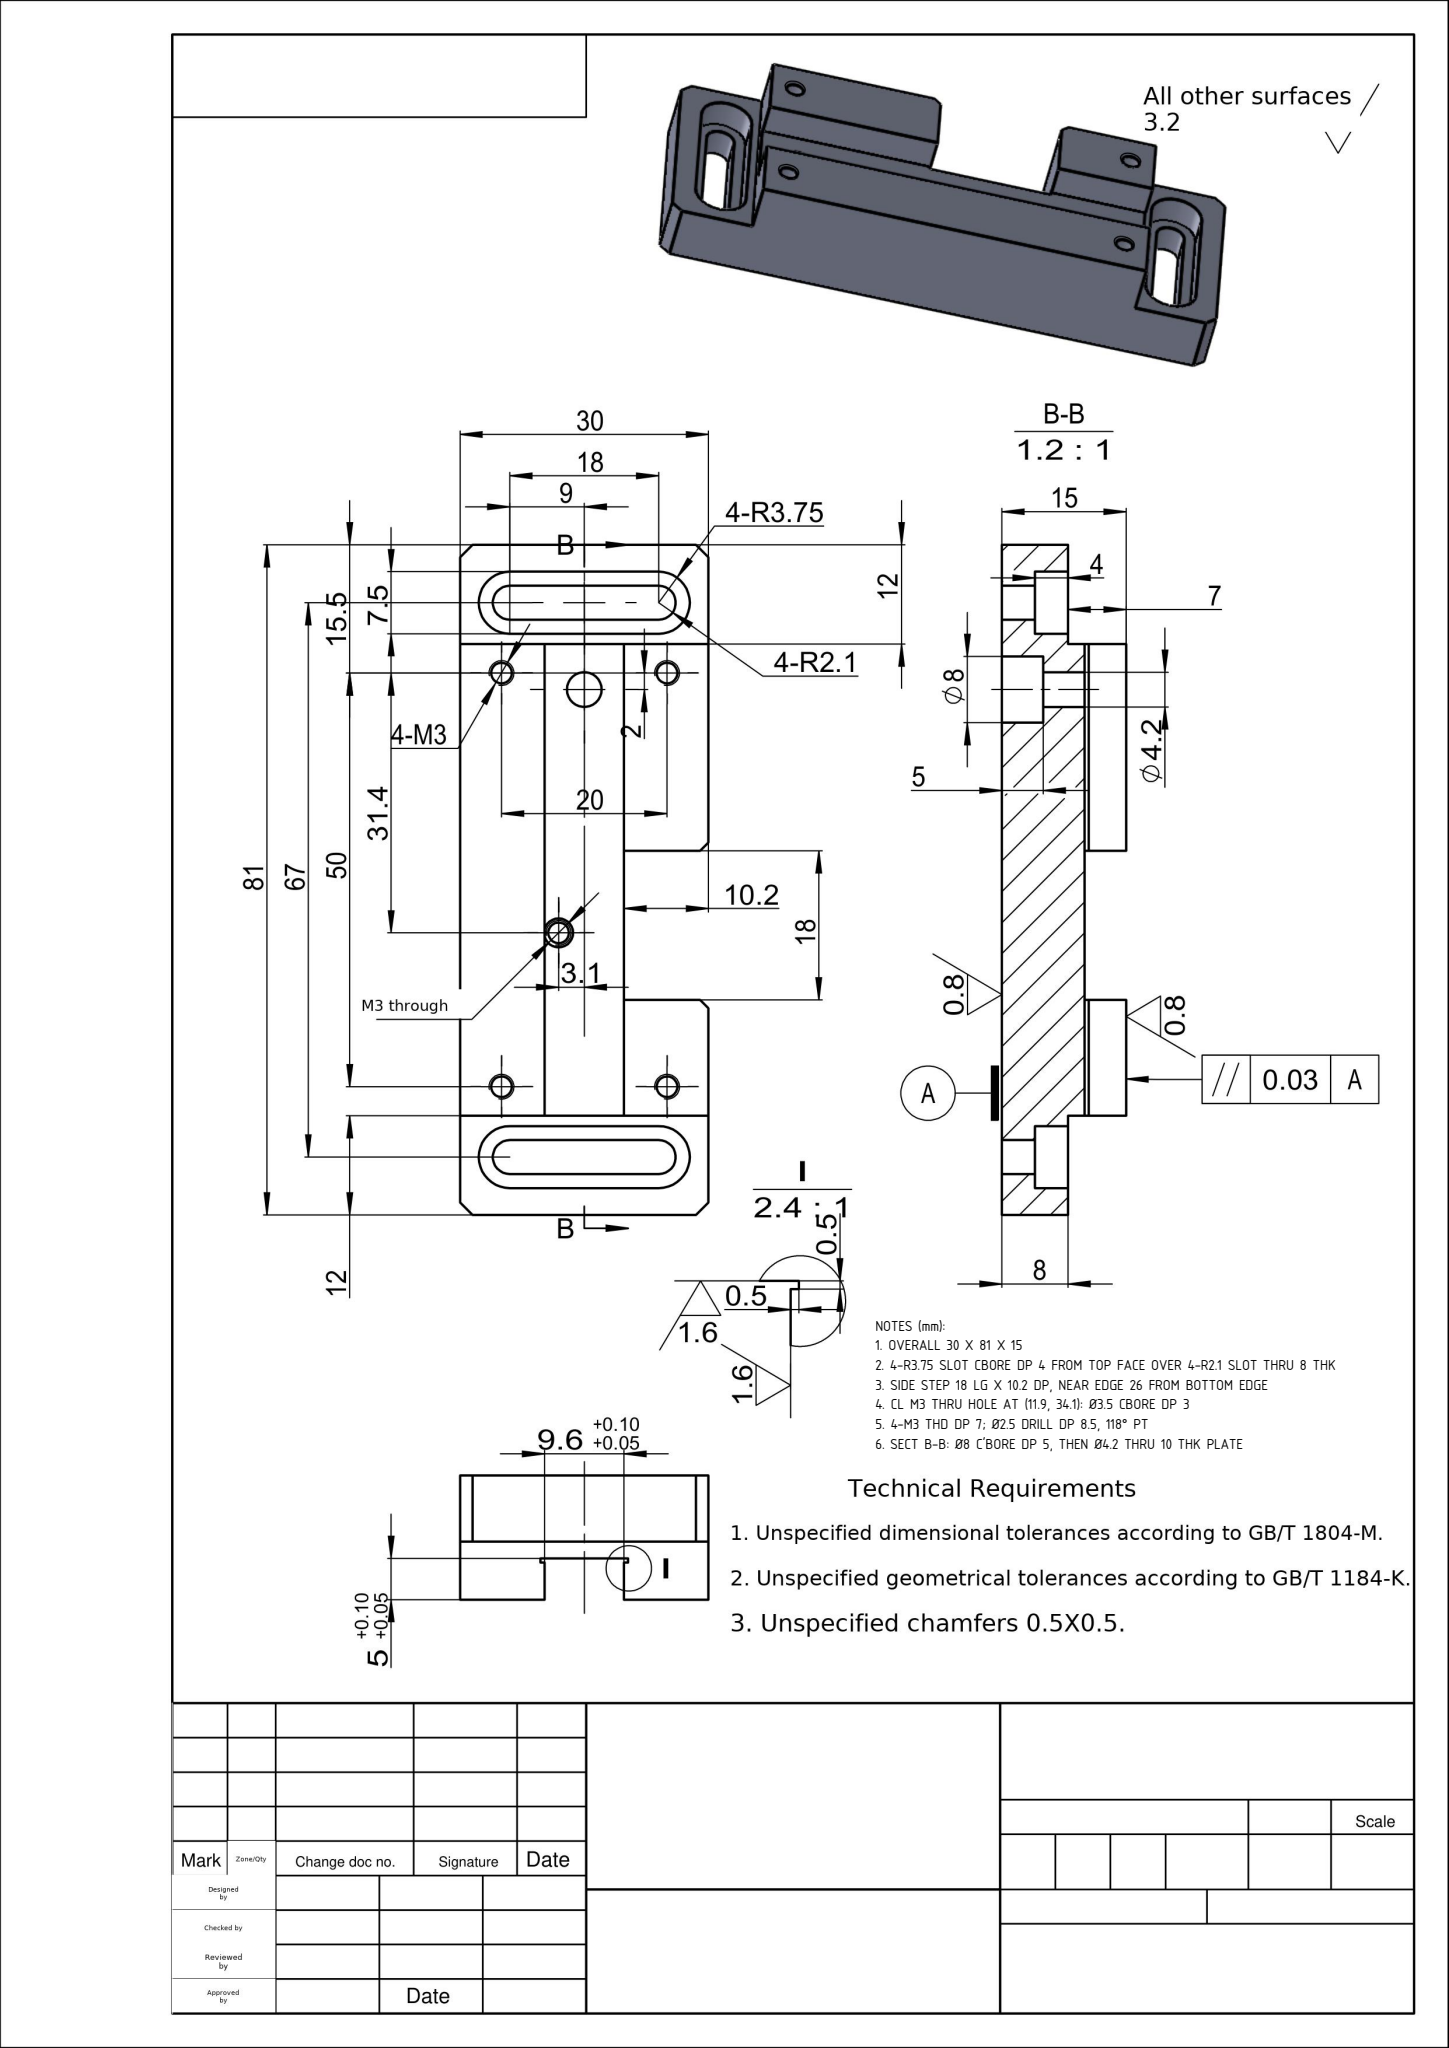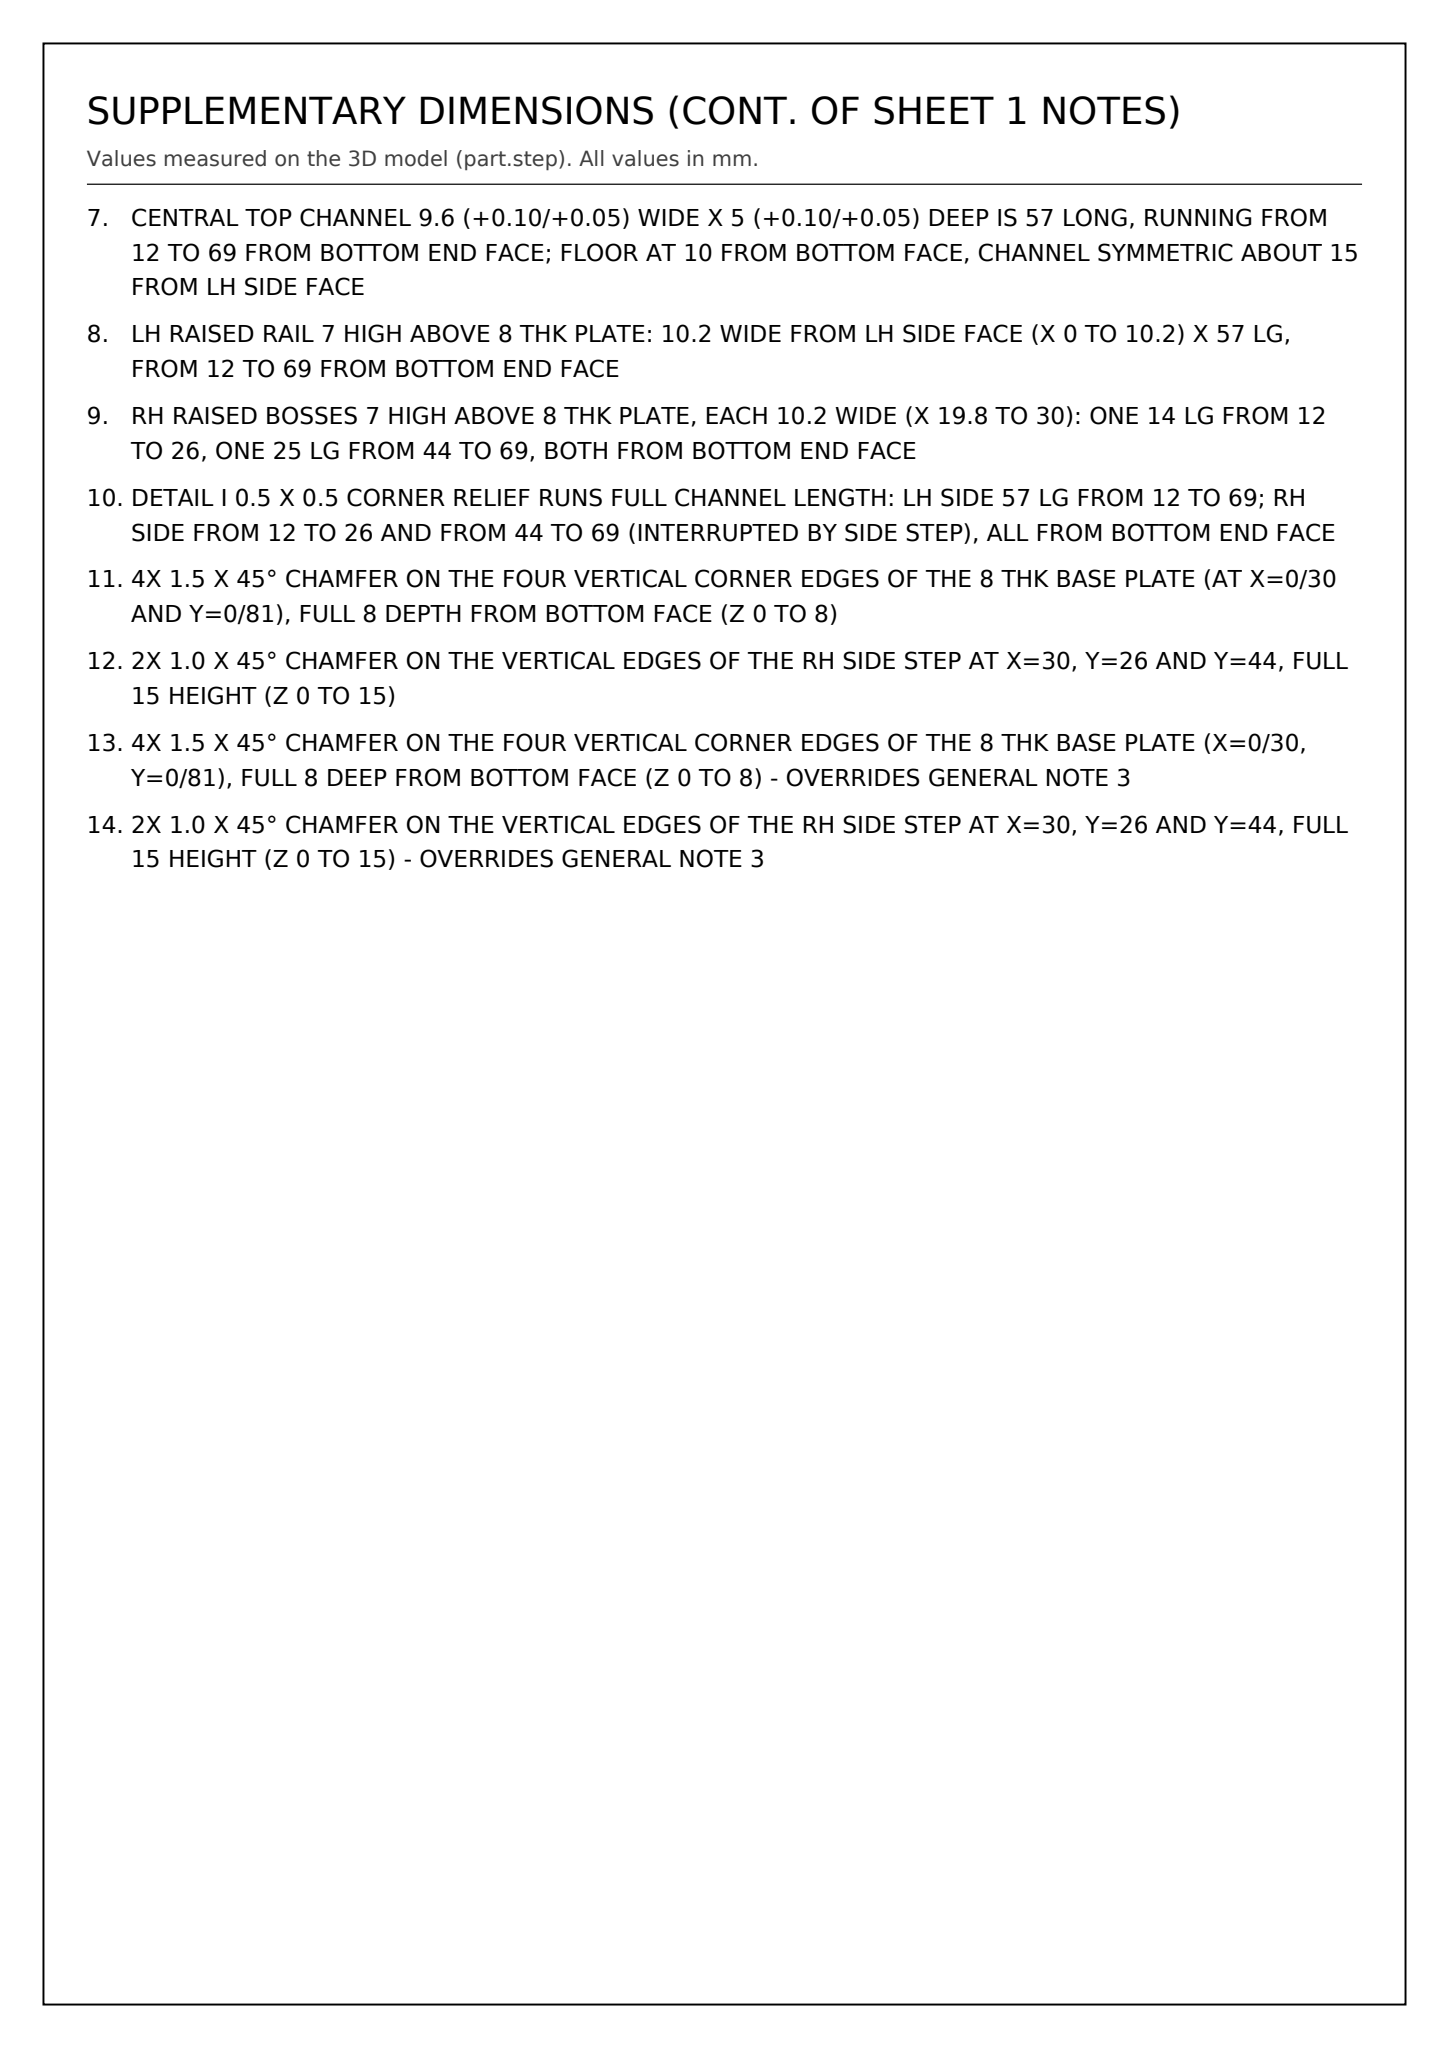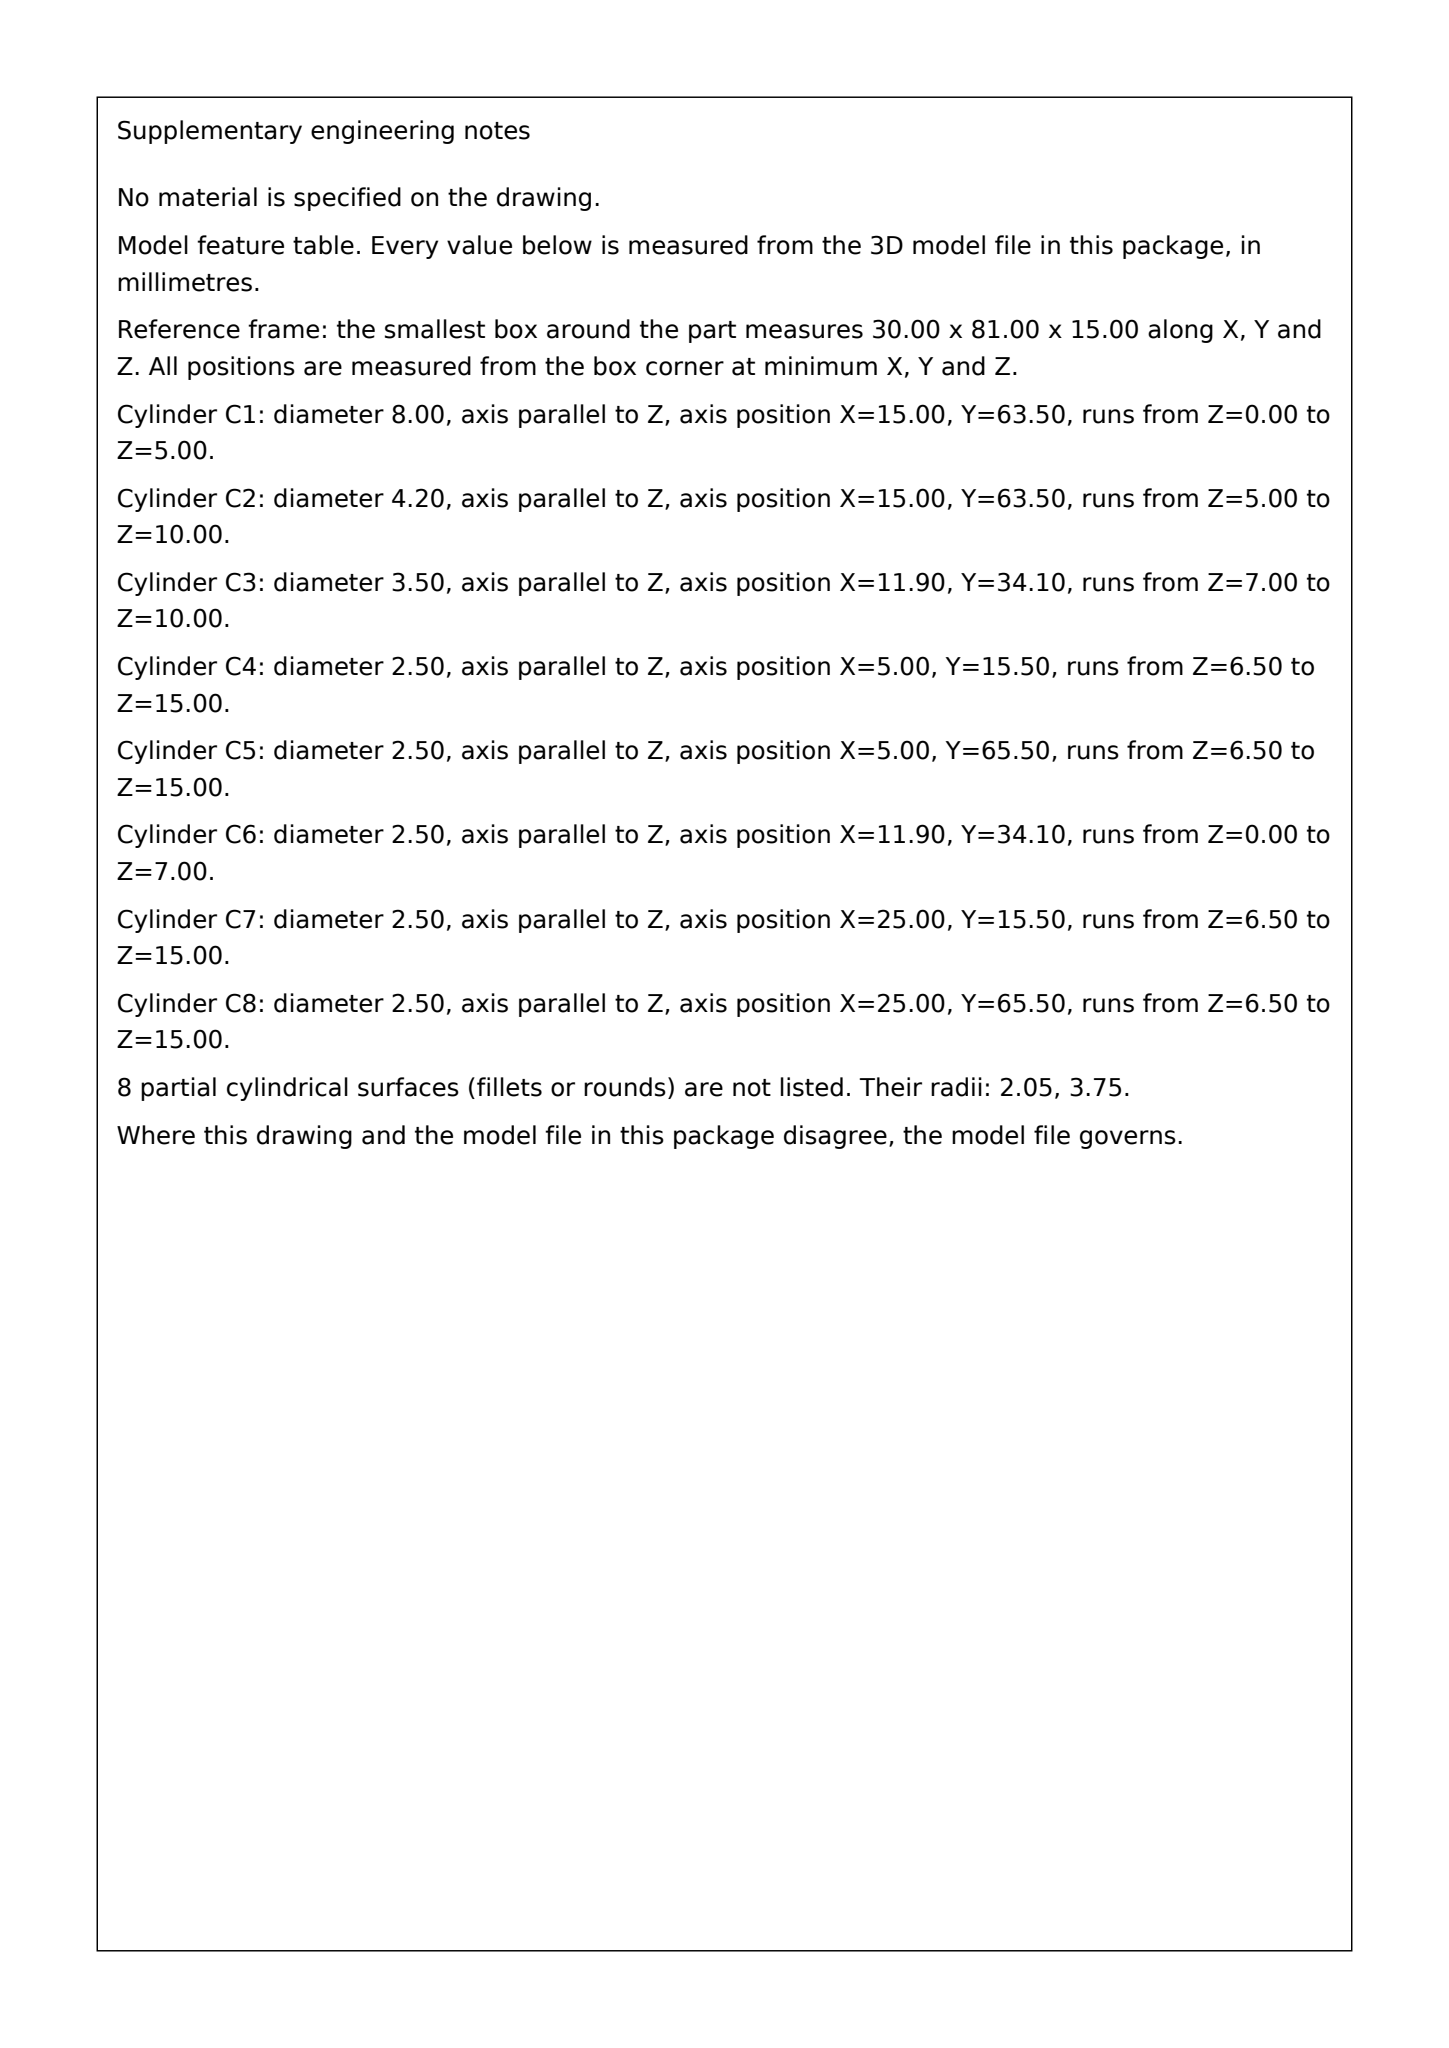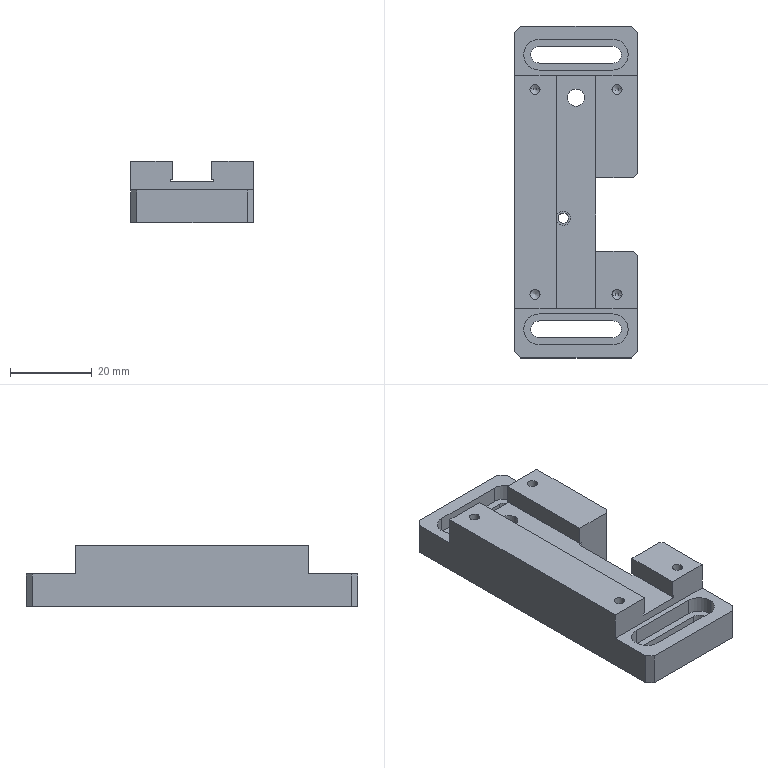Part | SolidWorks | mm | 1 solid | 80 faces | box 30 x 81 x 15 mm | volume 23160 mm3 | plane 44 | cylinder 28 | cone 8 | commonest cylinder face diameters 2.5 x10 4.1 x6 7.5 x6 3.5 x2 8 x2 4.2 x2
Drawing notes:
OVERALL 30 X 81 X 15 | from the solid: bbox_xyz [30.0, 81.0, 15.0]
4-R3.75 SLOT CBORE DP 4 FROM TOP FACE OVER 4-R2.1 SLOT THRU 8 THK | from the solid: Ø7.5 z-cyls L4.0 at (6,7),(6,74),(24,7),(24,74) over Ø4.1 z-cyls L4.0 same CL; z planes 15/10.5/7
SIDE STEP 18 LG X 10.2 DP, NEAR EDGE 26 FROM BOTTOM EDGE | from the solid: y planes 26.0 and 44.0 (18 apart) with x plane 10.2 forming notch; bbox y 0-81
CL M3 THRU HOLE AT (11.9, 34.1): Ø3.5 CBORE DP 3 | from the solid: coaxial Ø2.5 L7.0 and Ø3.5 L3.0 z-cyls at x=11.9, y=34.1; plate 10 thk
4-M3 THD DP 7; Ø2.5 DRILL DP 8.5, 118° PT | from the solid: Cylinders Ø2.5 z-axis at (5,15.5),(25,15.5),(5,65.5),(25,65.5), len 8.5; cone 118° ref dia 2.5
SECT B-B: Ø8 C'BORE DP 5, THEN Ø4.2 THRU 10 THK PLATE | from the solid: Ø8 z-cyl at (15,63.5) len 5.0 + Ø4.2 z-cyl same axis len 5.0; z planes 0 and 10 = 10 thk plate
CENTRAL TOP CHANNEL 9.6 (+0.10/+0.05) WIDE X 5 (+0.10/+0.05) DEEP IS 57 LONG, RUNNING FROM 12 TO 69 FROM BOTTOM END FACE; FLOOR AT 10 FROM BOTTOM FACE, CHANNEL SYMMETRIC ABOUT 15 FROM LH SIDE FACE | from the solid: axis_plane z=10 extent x[9.7,20.3] y[12,69]; axis_planes x=10.2 and x=19.8 z[10.5,15]; bounding faces y=12 and y=69 z[8,15]
LH RAISED RAIL 7 HIGH ABOVE 8 THK PLATE: 10.2 WIDE FROM LH SIDE FACE (X 0 TO 10.2) X 57 LG, FROM 12 TO 69 FROM BOTTOM END FACE | from the solid: axis_plane z=15 extent x[0,10.2] y[12,69]; axis_planes z=8 at y[0,12] and y[69,81]
RH RAISED BOSSES 7 HIGH ABOVE 8 THK PLATE, EACH 10.2 WIDE (X 19.8 TO 30): ONE 14 LG FROM 12 TO 26, ONE 25 LG FROM 44 TO 69, BOTH FROM BOTTOM END FACE | from the solid: axis_planes z=15 extent x[19.8,30] y[12,26] and x[19.8,30] y[44,69]
DETAIL I 0.5 X 0.5 CORNER RELIEF RUNS FULL CHANNEL LENGTH: LH SIDE 57 LG FROM 12 TO 69; RH SIDE FROM 12 TO 26 AND FROM 44 TO 69 (INTERRUPTED BY SIDE STEP), ALL FROM BOTTOM END FACE | from the solid: axis_planes z=10.5 extent x[9.7,10.2] y[12,69], x[19.8,20.3] y[12,26], x[19.8,20.3] y[44,69]
4X 1.5 X 45° CHAMFER ON THE FOUR VERTICAL CORNER EDGES OF THE 8 THK BASE PLATE (AT X=0/30 AND Y=0/81), FULL 8 DEPTH FROM BOTTOM FACE (Z 0 TO 8) | from the solid: inclined_planes: 4X angle 45/45/90, bbox_from [0,0,0], [0,79.5,0], [28.5,0,0], [28.5,79.5,0], size [1.5,1.5,8.0]
2X 1.0 X 45° CHAMFER ON THE VERTICAL EDGES OF THE RH SIDE STEP AT X=30, Y=26 AND Y=44, FULL 15 HEIGHT (Z 0 TO 15) | from the solid: inclined_planes: 2X angle 45/45/90, bbox_from [29.0,25.0,0.0] and [29.0,44.0,0.0], size [1.0,1.0,15.0]
4X 1.5 X 45° CHAMFER ON THE FOUR VERTICAL CORNER EDGES OF THE 8 THK BASE PLATE (X=0/30, Y=0/81), FULL 8 DEEP FROM BOTTOM FACE (Z 0 TO 8) - OVERRIDES GENERAL NOTE 3 | from the solid: inclined_planes: 4X angle_to_xyz_axes [45,45,90], size [1.5,1.5,8.0] at bbox_from [0,0,0], [0,79.5,0], [28.5,0,0], [28.5,79.5,0]
2X 1.0 X 45° CHAMFER ON THE VERTICAL EDGES OF THE RH SIDE STEP AT X=30, Y=26 AND Y=44, FULL 15 HEIGHT (Z 0 TO 15) - OVERRIDES GENERAL NOTE 3 | from the solid: inclined_planes: 2X angle_to_xyz_axes [45,45,90], size [1.0,1.0,15.0] at bbox_from [29.0,25.0,0] and [29.0,44.0,0]
build123d program:
from build123d import *

# Parameters (mm, degrees)
SKETCH1_W             = 30
SKETCH1_H             = 57
BOSS_EXTRUDE1_DEPTH   = 15
CUT_EXTRUDE1_REACH    = 68.136
M3_TAPPED_HOLE1_D     = 2.5
M3_TAPPED_HOLE1_DEPTH = 8.5
M3_TAPPED_HOLE1_TIP   = 0.7511
CUT_EXTRUDE2_REACH    = 67.184
SKETCH8_R             = 2.1
SKETCH9_R             = 4
CUT_EXTRUDE3_DEPTH    = 5
SKETCH11_R            = 1.75
CUT_EXTRUDE5_DEPTH    = 3
M3_TAPPED_HOLE2_D     = 2.5
SKETCH16_W            = 8
SKETCH16_H            = 57
BOSS_EXTRUDE2_DEPTH   = 70
CUT_EXTRUDE7_REACH    = 94.914
CHAMFER4_SIZE         = 40
CHAMFER4_SIZE2        = 20
CUT_EXTRUDE8_DEPTH    = 4.2
M4_TAPPED_HOLE1_D     = 3.3
M4_TAPPED_HOLE1_DEPTH = 11.5
M4_TAPPED_HOLE1_TIP   = 0.9914
SKETCH23_W            = 28.296
SKETCH23_H            = 76.025
CUT_EXTRUDE10_DEPTH   = 96.126
SKETCH24_W            = 10.2
SKETCH24_H            = 18
CUT_EXTRUDE11_DEPTH   = 67.136
CHAMFER5_SIZE         = 1
SKETCH25_W            = 30
SKETCH25_H            = 8
BOSS_EXTRUDE3_DEPTH   = 12
SKETCH26_W            = 30
SKETCH26_H            = 8
BOSS_EXTRUDE4_DEPTH   = 12
CUT_EXTRUDE12_DEPTH   = 4
CUT_EXTRUDE13_DEPTH   = 77.039
CHAMFER6_SIZE         = 1.5


with BuildPart() as part:
    # Sketch1 → Boss-Extrude1 (new body)
    with BuildSketch(Plane.XY):
        with Locations((15, -28.5)):
            Rectangle(SKETCH1_W, SKETCH1_H)
    extrude(amount=BOSS_EXTRUDE1_DEPTH)

    # Sketch2 → Cut-Extrude1 (cut, up to next)
    with BuildSketch(Plane.XZ.offset(57), mode=Mode.PRIVATE) as cut_extrude1_sk1:
        Polygon((10.2, 15), (19.8, 15), (19.8, 10.5), (20.3, 10.5), (20.3, 10), (19.8, 10), (9.7, 10), (9.7, 10.5), (10.2, 10.5), align=None)
    cut_extrude1_tool1 = extrude(cut_extrude1_sk1.sketch, amount=-CUT_EXTRUDE1_REACH, mode=Mode.PRIVATE) & part.part
    add(cut_extrude1_tool1.solids().sort_by_distance((15, -57, 12.477))[0], mode=Mode.SUBTRACT)

    # M3 Tapped Hole1
    with Locations(Plane.XY.offset(15)):
        with Locations((5, -3.5), (25, -3.5), (25, -53.5), (5, -53.5)):
            Hole(M3_TAPPED_HOLE1_D / 2, depth=M3_TAPPED_HOLE1_DEPTH)
            with Locations((0, 0, -(M3_TAPPED_HOLE1_DEPTH + M3_TAPPED_HOLE1_TIP / 2))):  # 118° drill point
                Cone(0, M3_TAPPED_HOLE1_D / 2, M3_TAPPED_HOLE1_TIP, mode=Mode.SUBTRACT)

    # Sketch8 → Cut-Extrude2 (cut, up to next)
    with BuildSketch(Plane.XY.offset(10), mode=Mode.PRIVATE) as cut_extrude2_sk1:
        with Locations((15, -5.5)):
            Circle(SKETCH8_R)
    cut_extrude2_tool1 = extrude(cut_extrude2_sk1.sketch, amount=-CUT_EXTRUDE2_REACH, mode=Mode.PRIVATE) & part.part
    add(cut_extrude2_tool1.solids().sort_by_distance((15, -5.5, 10))[0], mode=Mode.SUBTRACT)

    # Sketch9 → Cut-Extrude3 (cut)
    with BuildSketch(Plane(origin=(0, 0, 0), x_dir=(-1, 0, 0), z_dir=(0, 0, -1))):
        with Locations((-15, -5.5)):
            Circle(SKETCH9_R)
    extrude(amount=-CUT_EXTRUDE3_DEPTH, mode=Mode.SUBTRACT)

    # Sketch11 → Cut-Extrude5 (cut)
    with BuildSketch(Plane.XY.offset(10)):
        with Locations((11.9, -34.9)):
            Circle(SKETCH11_R)
    extrude(amount=-CUT_EXTRUDE5_DEPTH, mode=Mode.SUBTRACT)

    # M3 Tapped Hole2 (through all)
    with Locations(Plane.XY.offset(7)):
        with Locations((11.9, -34.9)):
            Hole(M3_TAPPED_HOLE2_D / 2)

    # Sketch16 → Boss-Extrude2 (add)
    with BuildSketch(Plane(origin=(0, 0, 0), x_dir=(-1, 0, 0), z_dir=(0, 0, -1))):
        with Locations((-26, -28.5)):
            Rectangle(SKETCH16_W, SKETCH16_H)
    extrude(amount=BOSS_EXTRUDE2_DEPTH)

    # Sketch18 → Cut-Extrude7 (cut, up to next)
    with BuildSketch(Plane.ZY.offset(-22), mode=Mode.PRIVATE) as cut_extrude7_sk1:
        with BuildLine():
            Line((-60, -4.4), (-55, -4.4))
            ThreePointArc((-55, -4.4), (-52.9, -6.5), (-55, -8.6))
            Line((-55, -8.6), (-60, -8.6))
            ThreePointArc((-60, -8.6), (-62.1, -6.5), (-60, -4.4))
        make_face()
    cut_extrude7_tool1 = extrude(cut_extrude7_sk1.sketch, amount=-CUT_EXTRUDE7_REACH, mode=Mode.PRIVATE) & part.part
    # Sketch18 → Cut-Extrude7 (cut, up to next)
    with BuildSketch(Plane.ZY.offset(-22), mode=Mode.PRIVATE) as cut_extrude7_sk2:
        with BuildLine():
            Line((-30, -4.4), (-35, -4.4))
            ThreePointArc((-35, -4.4), (-37.1, -6.5), (-35, -8.6))
            Line((-35, -8.6), (-30, -8.6))
            ThreePointArc((-30, -8.6), (-27.9, -6.5), (-30, -4.4))
        make_face()
    cut_extrude7_tool2 = extrude(cut_extrude7_sk2.sketch, amount=-CUT_EXTRUDE7_REACH, mode=Mode.PRIVATE) & part.part
    # Sketch18 → Cut-Extrude7 (cut, up to next)
    with BuildSketch(Plane.ZY.offset(-22), mode=Mode.PRIVATE) as cut_extrude7_sk3:
        with BuildLine():
            Line((-30, -28.6), (-35, -28.6))
            ThreePointArc((-35, -28.6), (-37.1, -26.5), (-35, -24.4))
            Line((-35, -24.4), (-30, -24.4))
            ThreePointArc((-30, -24.4), (-27.9, -26.5), (-30, -28.6))
        make_face()
    cut_extrude7_tool3 = extrude(cut_extrude7_sk3.sketch, amount=-CUT_EXTRUDE7_REACH, mode=Mode.PRIVATE) & part.part
    # Sketch18 → Cut-Extrude7 (cut, up to next)
    with BuildSketch(Plane.ZY.offset(-22), mode=Mode.PRIVATE) as cut_extrude7_sk4:
        with BuildLine():
            Line((-60, -28.6), (-55, -28.6))
            ThreePointArc((-55, -28.6), (-52.9, -26.5), (-55, -24.4))
            Line((-55, -24.4), (-60, -24.4))
            ThreePointArc((-60, -24.4), (-62.1, -26.5), (-60, -28.6))
        make_face()
    cut_extrude7_tool4 = extrude(cut_extrude7_sk4.sketch, amount=-CUT_EXTRUDE7_REACH, mode=Mode.PRIVATE) & part.part
    add(cut_extrude7_tool1.solids().sort_by_distance((22, -6.5, -57.5))[0], mode=Mode.SUBTRACT)
    add(cut_extrude7_tool2.solids().sort_by_distance((22, -6.5, -32.5))[0], mode=Mode.SUBTRACT)
    add(cut_extrude7_tool3.solids().sort_by_distance((22, -26.5, -32.5))[0], mode=Mode.SUBTRACT)
    add(cut_extrude7_tool4.solids().sort_by_distance((22, -26.5, -57.5))[0], mode=Mode.SUBTRACT)

    # Chamfer4
    chamfer4_edges = [part.edges().sort_by_distance(p)[0] for p in [
        (26, -57, -70),
    ]]
    chamfer4_side = [part.faces().sort_by_distance(p)[0] for p in [
        (11, -57, 0.9014),
    ]]
    chamfer(chamfer4_edges, length=CHAMFER4_SIZE, length2=CHAMFER4_SIZE2, reference=chamfer4_side[0])

    # Sketch19 → Cut-Extrude8 (cut)
    with BuildSketch(Plane.ZY.offset(-22)):
        with BuildLine():
            Line((-60, -2.5), (-55, -2.5))
            ThreePointArc((-55, -2.5), (-51, -6.5), (-55, -10.5))
            Line((-55, -10.5), (-60, -10.5))
            ThreePointArc((-60, -10.5), (-64, -6.5), (-60, -2.5))
        make_face()
        with BuildLine():
            Line((-35, -2.5), (-30, -2.5))
            ThreePointArc((-30, -2.5), (-26, -6.5), (-30, -10.5))
            Line((-30, -10.5), (-35, -10.5))
            ThreePointArc((-35, -10.5), (-39, -6.5), (-35, -2.5))
        make_face()
        with BuildLine():
            Line((-60, -22.5), (-55, -22.5))
            ThreePointArc((-55, -22.5), (-51, -26.5), (-55, -30.5))
            Line((-55, -30.5), (-60, -30.5))
            ThreePointArc((-60, -30.5), (-64, -26.5), (-60, -22.5))
        make_face()
        with BuildLine():
            Line((-35, -22.5), (-30, -22.5))
            ThreePointArc((-30, -22.5), (-26, -26.5), (-30, -30.5))
            Line((-30, -30.5), (-35, -30.5))
            ThreePointArc((-35, -30.5), (-39, -26.5), (-35, -22.5))
        make_face()
    extrude(amount=-CUT_EXTRUDE8_DEPTH, mode=Mode.SUBTRACT)

    # M4 Tapped Hole1
    with Locations(Plane.ZY.offset(-22)):
        with Locations((-6, -16.5), (-26, -16.5)):
            Hole(M4_TAPPED_HOLE1_D / 2, depth=M4_TAPPED_HOLE1_DEPTH)
            with Locations((0, 0, -(M4_TAPPED_HOLE1_DEPTH + M4_TAPPED_HOLE1_TIP / 2))):  # 118° drill point
                Cone(0, M4_TAPPED_HOLE1_D / 2, M4_TAPPED_HOLE1_TIP, mode=Mode.SUBTRACT)

    # Sketch23 → Cut-Extrude10 (cut, through all)
    with BuildSketch(Plane(origin=(0, 0, 0), x_dir=(1, 0, 0), z_dir=(0, 1, 0))):
        with Locations((25.64, 38.012)):
            Rectangle(SKETCH23_W, SKETCH23_H)
    extrude(amount=-CUT_EXTRUDE10_DEPTH, mode=Mode.SUBTRACT)

    # Sketch24 → Cut-Extrude11 (cut, through all)
    with BuildSketch(Plane.XY.offset(15)):
        with Locations((24.9, -34)):
            Rectangle(SKETCH24_W, SKETCH24_H)
    extrude(amount=-CUT_EXTRUDE11_DEPTH, mode=Mode.SUBTRACT)

    # Chamfer5
    chamfer5_edges = [part.edges().sort_by_distance(p)[0] for p in [
        (30, -43, 7.5),
        (30, -25, 7.5),
    ]]
    chamfer(chamfer5_edges, length=CHAMFER5_SIZE)

    # Sketch25 → Boss-Extrude3 (add)
    with BuildSketch(Plane.XZ.offset(57)):
        with Locations((15, 4)):
            Rectangle(SKETCH25_W, SKETCH25_H)
    extrude(amount=BOSS_EXTRUDE3_DEPTH)

    # Sketch26 → Boss-Extrude4 (add)
    with BuildSketch(Plane(origin=(0, 0, 0), x_dir=(1, 0, 0), z_dir=(0, 1, 0))):
        with Locations((15, -4)):
            Rectangle(SKETCH26_W, SKETCH26_H)
    extrude(amount=BOSS_EXTRUDE4_DEPTH)

    # Sketch27 → Cut-Extrude12 (cut)
    with BuildSketch(Plane.XY.offset(8)):
        with BuildLine():
            Line((6, 8.75), (24, 8.75))
            ThreePointArc((24, 8.75), (27.75, 5), (24, 1.25))
            Line((24, 1.25), (6, 1.25))
            ThreePointArc((6, 1.25), (2.25, 5), (6, 8.75))
        make_face()
        with BuildLine():
            Line((6, -65.75), (24, -65.75))
            ThreePointArc((24, -65.75), (27.75, -62), (24, -58.25))
            Line((24, -58.25), (6, -58.25))
            ThreePointArc((6, -58.25), (2.25, -62), (6, -65.75))
        make_face()
    extrude(amount=-CUT_EXTRUDE12_DEPTH, mode=Mode.SUBTRACT)

    # Sketch28 → Cut-Extrude13 (cut, through all)
    with BuildSketch(Plane.XY.offset(4)):
        with BuildLine():
            Line((6, 7.05), (24, 7.05))
            ThreePointArc((24, 7.05), (26.05, 5), (24, 2.95))
            Line((24, 2.95), (6, 2.95))
            ThreePointArc((6, 2.95), (3.95, 5), (6, 7.05))
        make_face()
        with BuildLine():
            Line((6, -59.95), (24, -59.95))
            ThreePointArc((24, -59.95), (26.05, -62), (24, -64.05))
            Line((24, -64.05), (6, -64.05))
            ThreePointArc((6, -64.05), (3.95, -62), (6, -59.95))
        make_face()
    extrude(amount=-CUT_EXTRUDE13_DEPTH, mode=Mode.SUBTRACT)

    # Chamfer6
    chamfer6_edges = [part.edges().sort_by_distance(p)[0] for p in [
        (0, 12, 4),
        (30, 12, 4),
        (0, -69, 4),
        (30, -69, 4),
    ]]
    chamfer(chamfer6_edges, length=CHAMFER6_SIZE)


solid = part.part